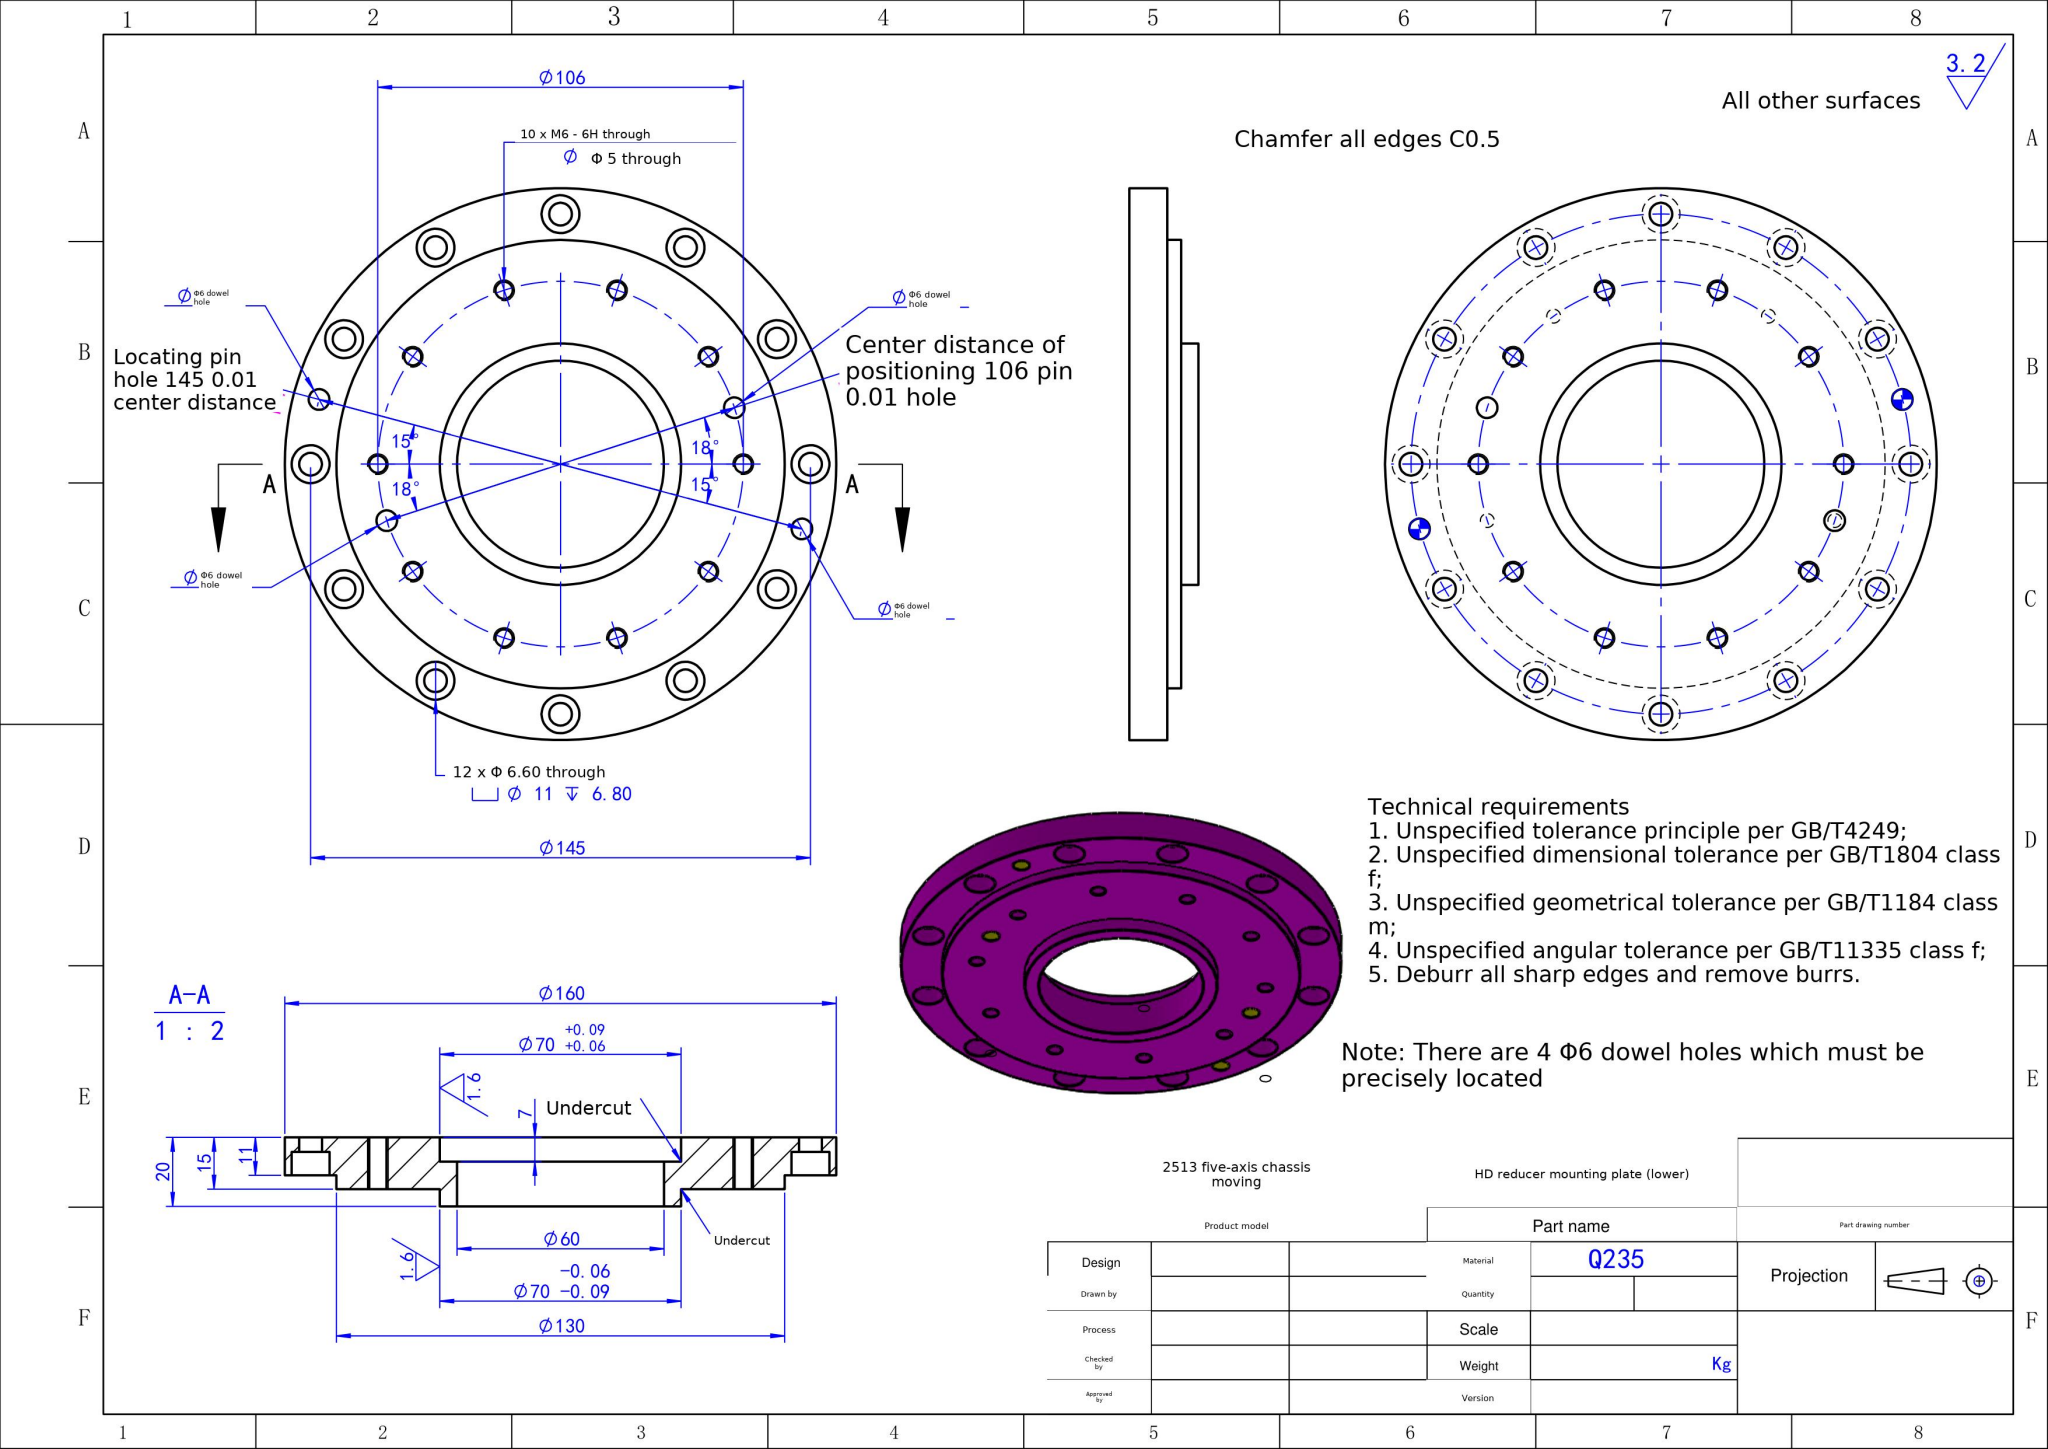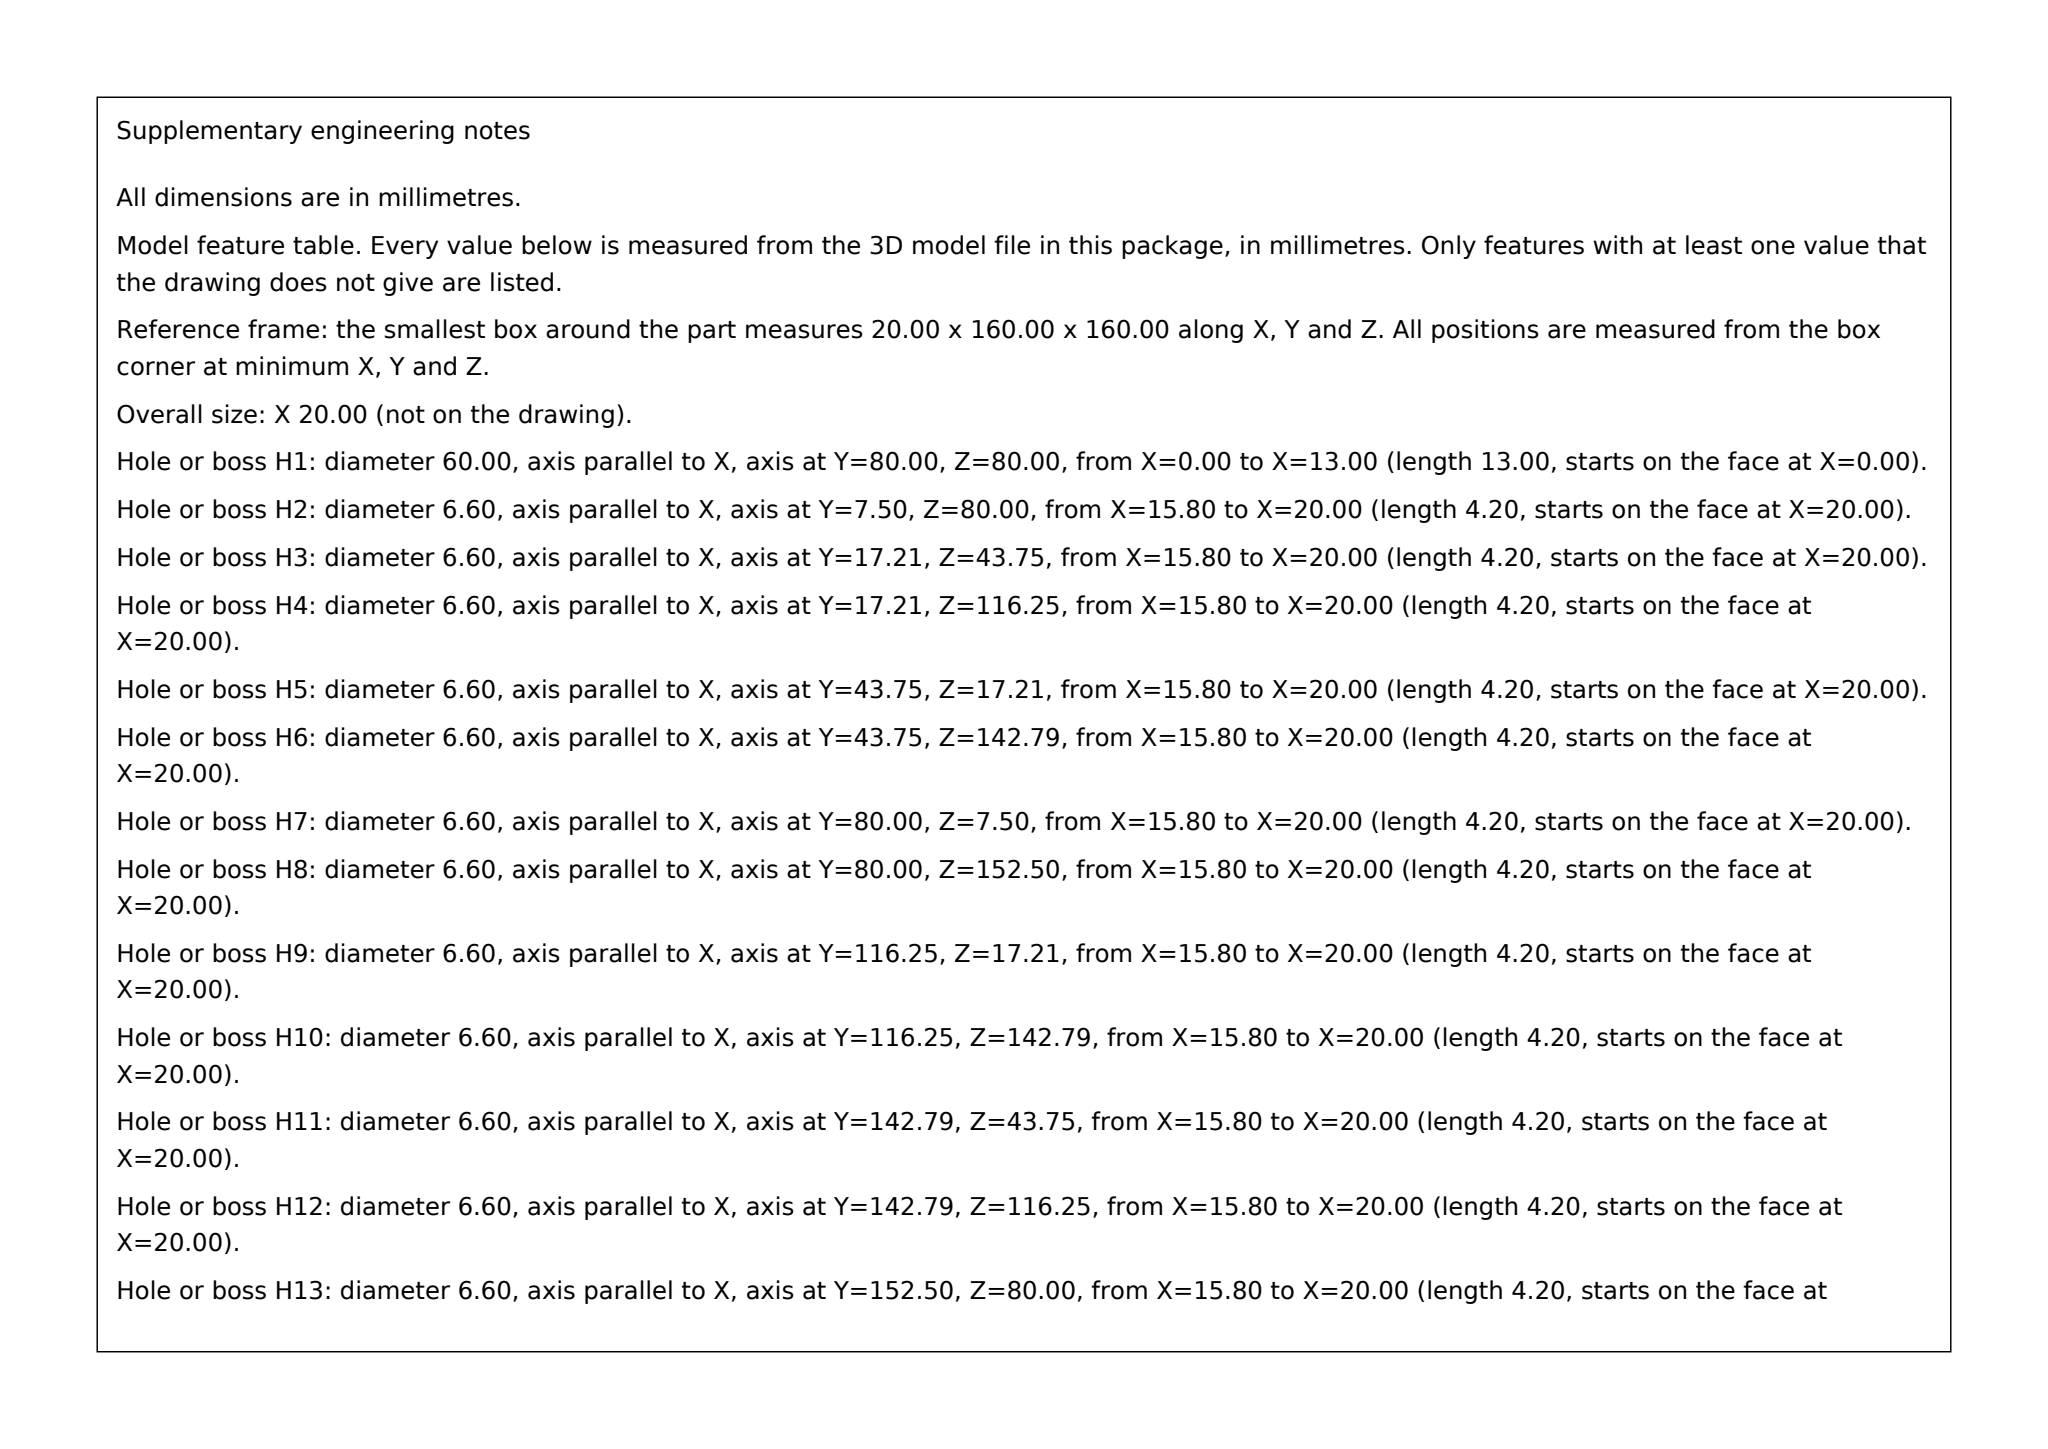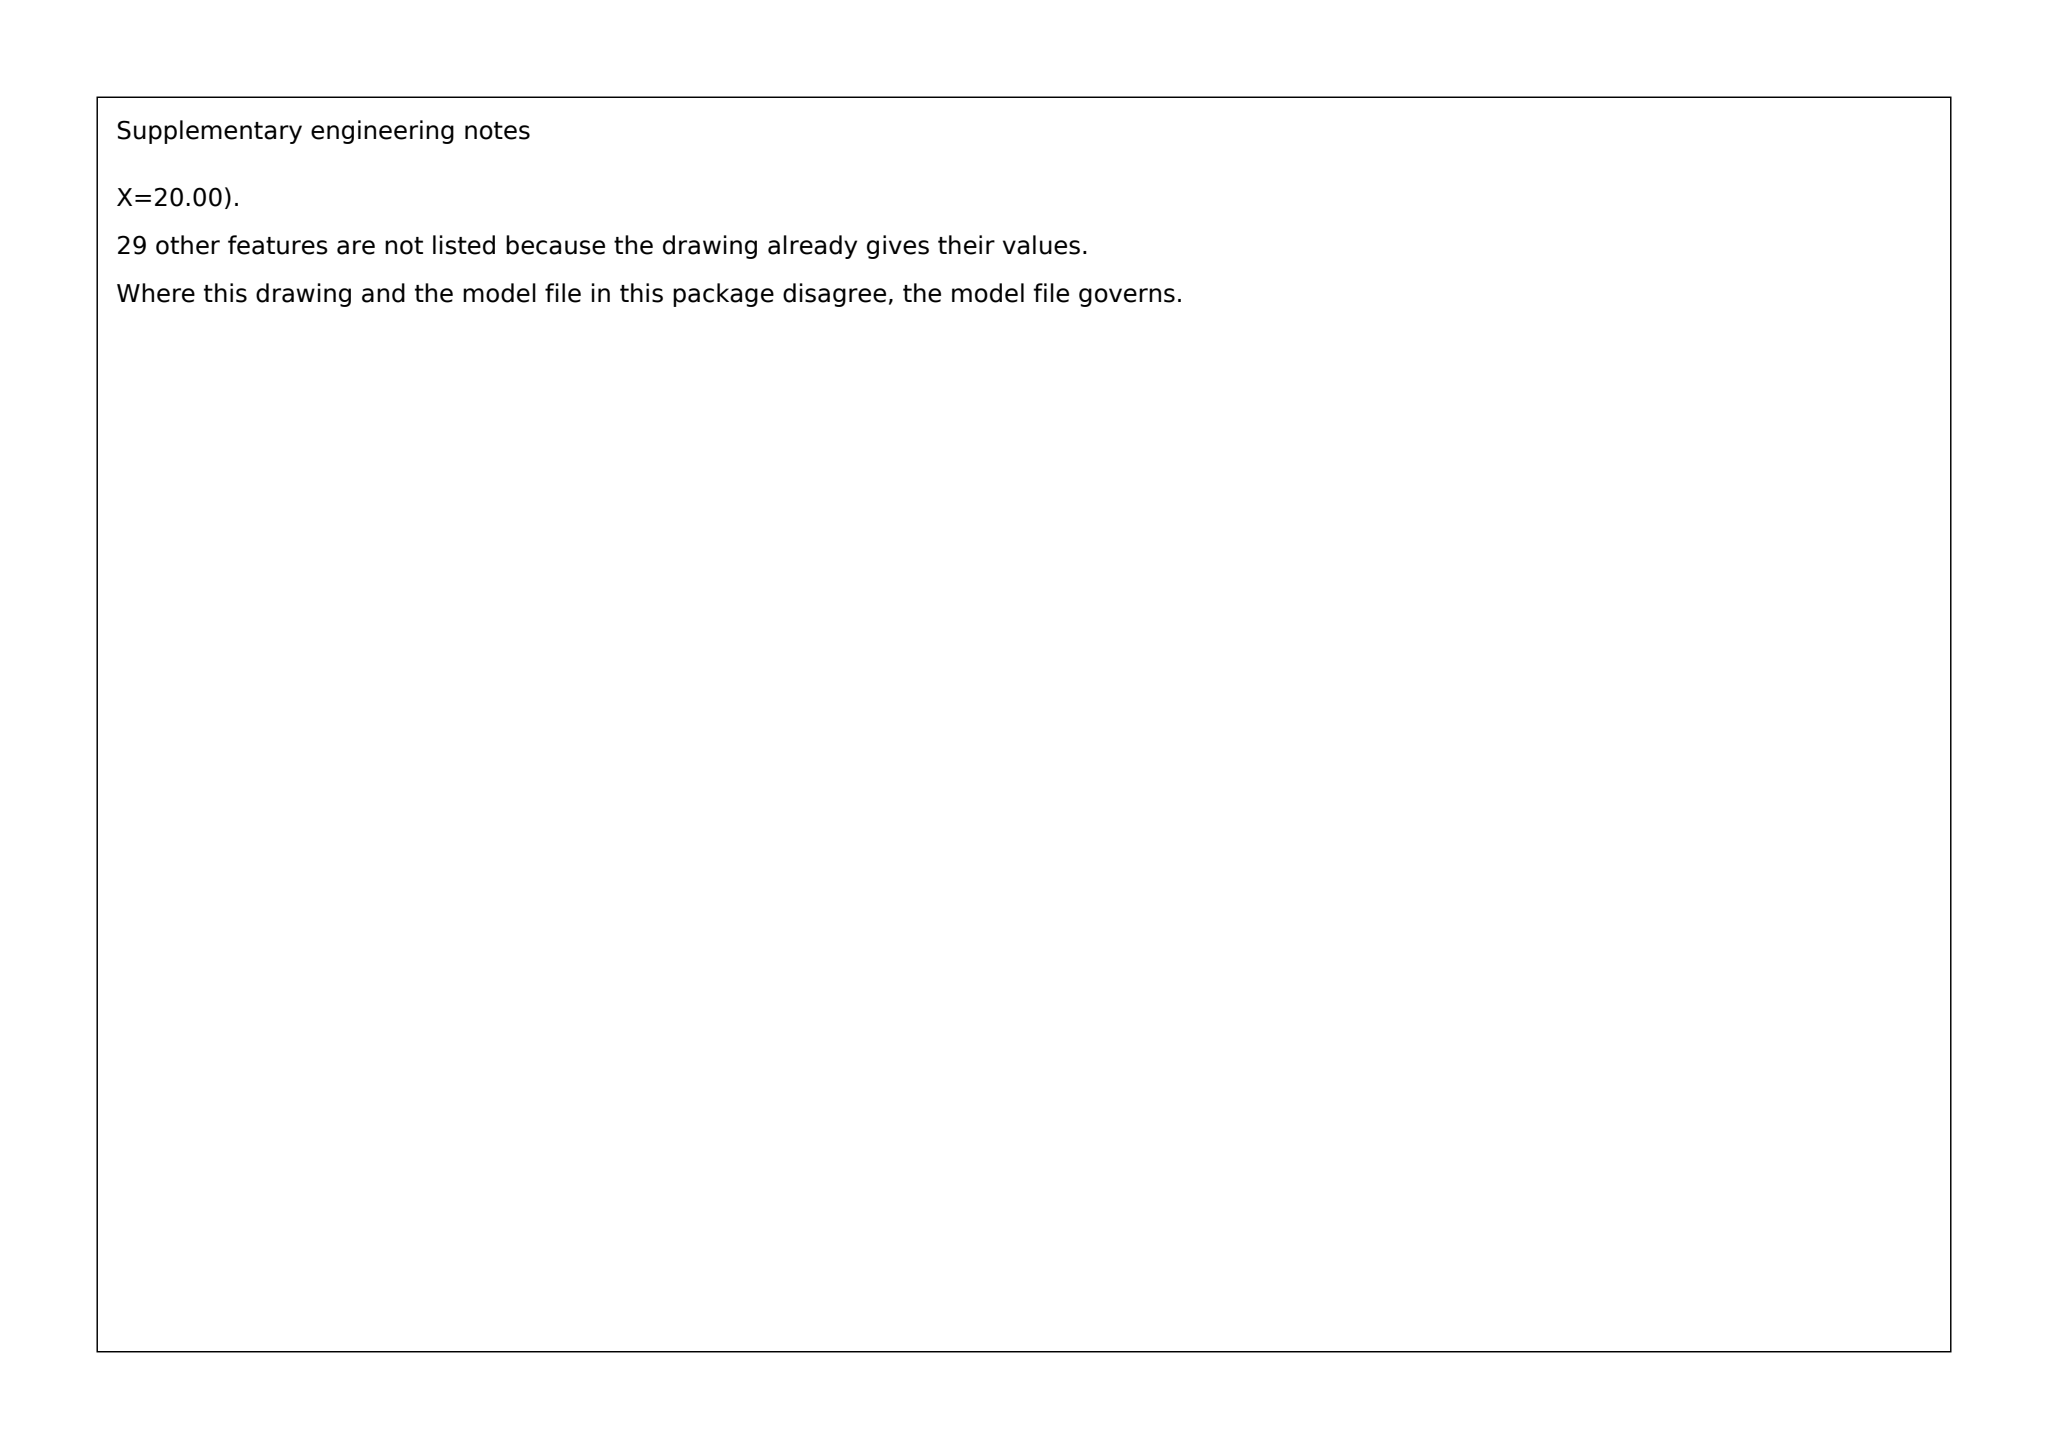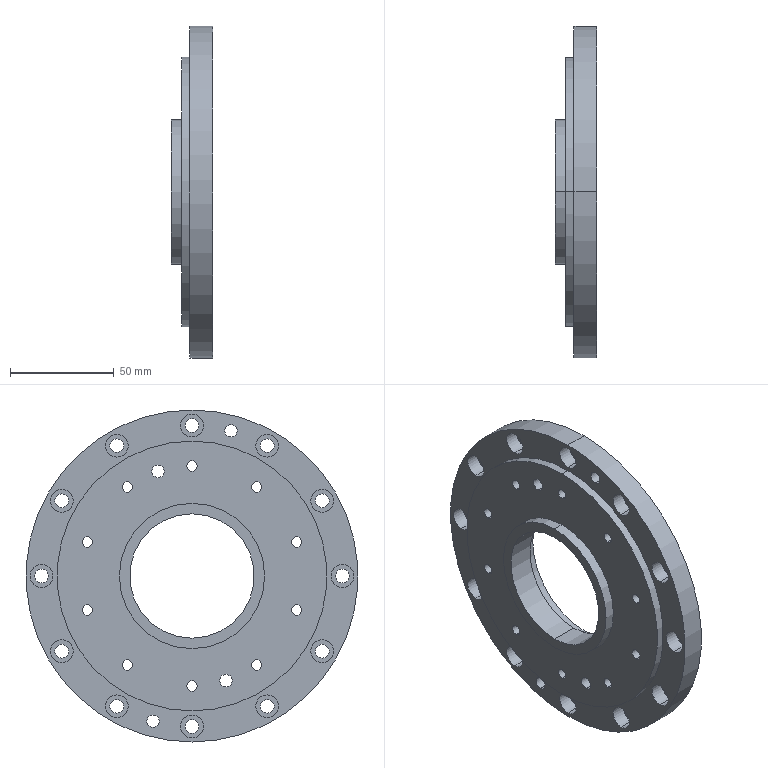Part | SolidWorks | mm | material Q235 | 1 solid | 103 faces | box 20 x 160 x 160 mm | volume 215913 mm3 | cylinder 86 | plane 17 | commonest cylinder face diameters 11 x24 6.6 x24 5 x20 6 x8 70 x4 160 x2 60 x2 130 x2